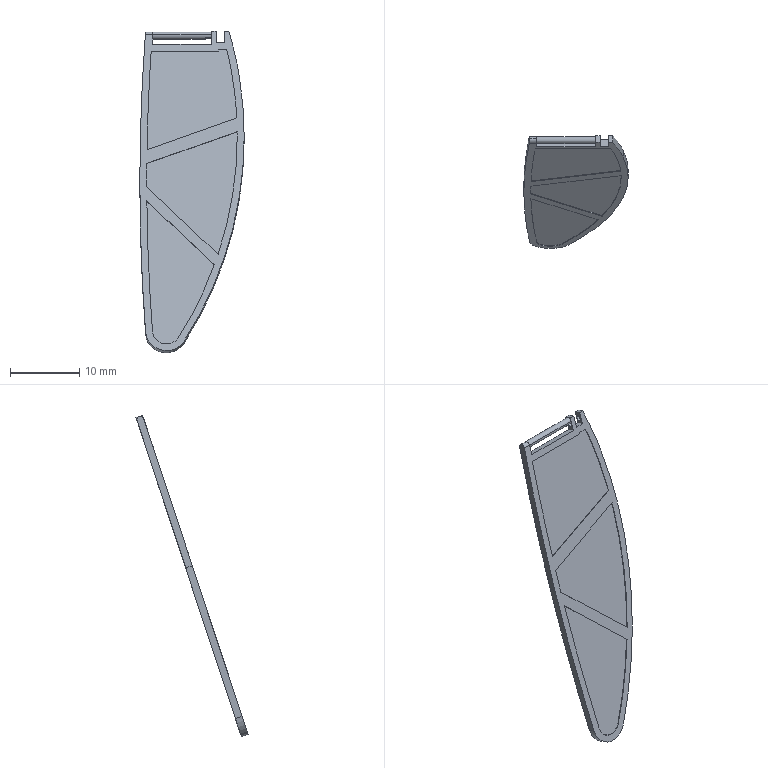Component | SolidWorks | RearWing-5 | 1 solid | 65 faces | volume 503 mm3 | plane 34 | cylinder 31 | commonest cylinder face diameters 118 x7 625.039 x7 0.8 x4 1 x4 627.039 x2 4 x2 108 x2 6 x1